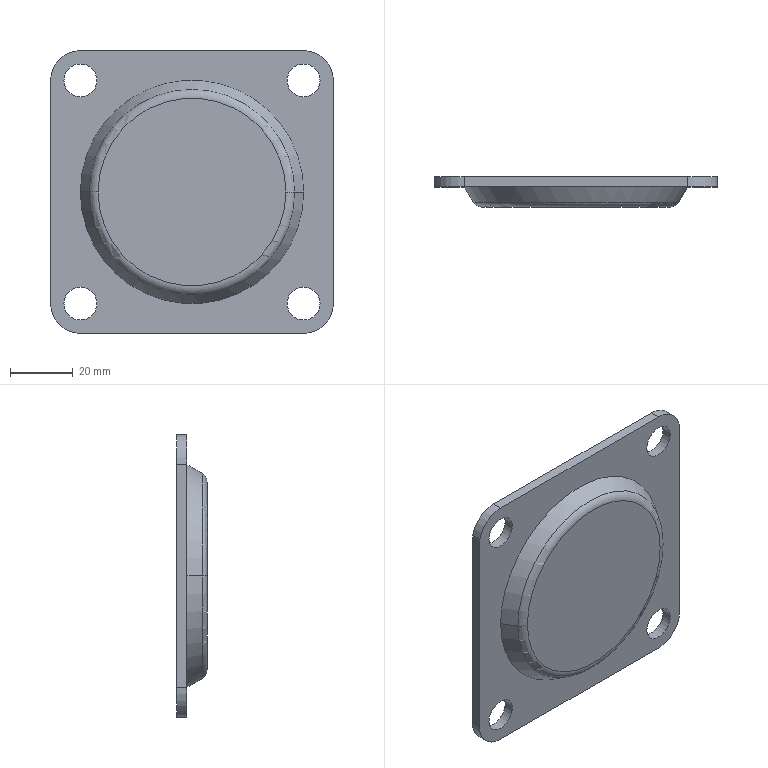Component | SolidWorks | 30-01A-1_Wheel-322-1_CJH65-322-1_CJH65swivel-322-1 | 1 solid | 47 faces | box 90 x 9.6 x 90 mm | volume 43061 mm3 | cylinder 18 | torus 16 | plane 11 | cone 2 | commonest cylinder face diameters 10.5 x8 19 x4 59 x2 30.5 x2 10 x2
build123d program:
from build123d import *

# Parameters (mm, degrees)
SKETCH1_R      = 5.25
EXTRUDE1_DEPTH = 3.2


with BuildPart() as part:
    # Sketch1 → Extrude1 (new body)
    with BuildSketch(Plane(origin=(0, 0, 0), x_dir=(1, 0, 0), z_dir=(0, 1, 0))):
        with BuildLine():
            Line((-35.5, -45), (35.5, -45))
            ThreePointArc((35.5, -45), (42.218, -42.218), (45, -35.5))
            Line((45, -35.5), (45, 35.5))
            ThreePointArc((45, 35.5), (42.218, 42.218), (35.5, 45))
            Line((35.5, 45), (-35.5, 45))
            ThreePointArc((-35.5, 45), (-42.218, 42.218), (-45, 35.5))
            Line((-45, 35.5), (-45, -35.5))
            ThreePointArc((-45, -35.5), (-42.218, -42.218), (-35.5, -45))
        make_face()
        with Locations(Location((35.5, -35.5, 0), (0, 0, 270))):
            Circle(SKETCH1_R, mode=Mode.SUBTRACT)
        with Locations(Location((35.5, 35.5, 0), (0, 0, 270))):
            Circle(SKETCH1_R, mode=Mode.SUBTRACT)
        with Locations(Location((-35.5, -35.5, 0), (0, 0, 270))):
            Circle(SKETCH1_R, mode=Mode.SUBTRACT)
        with Locations(Location((-35.5, 35.5, 0), (0, 0, 270))):
            Circle(SKETCH1_R, mode=Mode.SUBTRACT)
    extrude(amount=-EXTRUDE1_DEPTH)

    # Sketch2 → Revolve1 (revolve)
    with BuildSketch(Plane.XY, mode=Mode.PRIVATE) as revolve1_sk:
        with BuildLine():
            Line((0, -3.2), (35.5, -3.2))
            Line((35.5, -3.2), (32.598, -8.044))
            ThreePointArc((32.598, -8.044), (31.431, -9.184), (29.853, -9.6))
            Line((29.853, -9.6), (0, -9.6))
            Line((0, -9.6), (0, -3.2))
        make_face()
    revolve(revolve1_sk.sketch.rotate(Axis((0, -9.6, 0), (0, 1, 0)), 270), axis=Axis((0, -9.6, 0), (0, 1, 0)))

    # Sketch3 → Cut-Revolve1 (revolve, cut)
    with BuildSketch(Plane.XY, mode=Mode.PRIVATE) as cut_revolve1_sk:
        with BuildLine():
            Line((0, 0), (30.5, 0))
            ThreePointArc((30.5, 0), (29.793, -0.2929), (29.5, -1))
            Line((29.5, -1), (29.5, -1.5))
            ThreePointArc((29.5, -1.5), (29.354, -1.854), (29, -2))
            Line((29, -2), (27, -2))
            ThreePointArc((27, -2), (26.646, -1.854), (26.5, -1.5))
            ThreePointArc((26.5, -1.5), (26.207, -0.7929), (25.5, -0.5))
            Line((25.5, -0.5), (16.25, -0.5))
            ThreePointArc((16.25, -0.5), (15.543, -0.7929), (15.25, -1.5))
            Line((15.25, -1.5), (15.25, -2.2))
            ThreePointArc((15.25, -2.2), (14.957, -2.907), (14.25, -3.2))
            Line((14.25, -3.2), (5, -3.2))
            Line((5, -3.2), (5, -3))
            ThreePointArc((5, -3), (4.707, -2.293), (4, -2))
            Line((4, -2), (0, -2))
            Line((0, -2), (0, 0))
        make_face()
    revolve(cut_revolve1_sk.sketch.rotate(Axis((0, -2, 0), (0, 1, 0)), 270), axis=Axis((0, -2, 0), (0, 1, 0)), mode=Mode.SUBTRACT)


solid = part.part

# Placed as in the assembly
solid = solid.moved(Location((158.07, -562.845, -114.5), (0, 0, 0)))